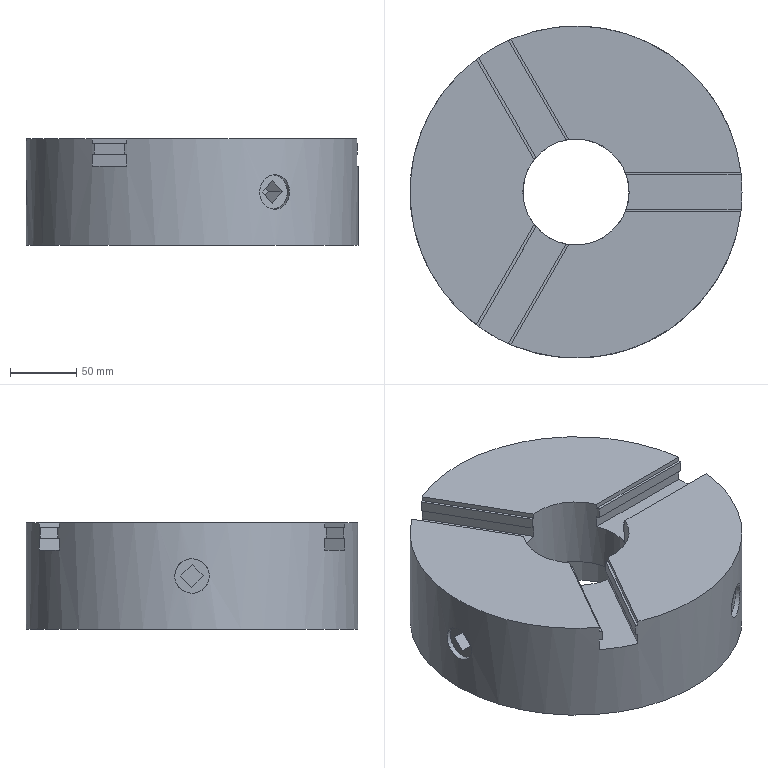Component | NX | Root-owned geometry | 1 solid | 69 faces | volume 3258312 mm3 | plane 59 | cylinder 10 | commonest cylinder face diameters 26 x3 18 x3 80 x2 250 x1 103 x1